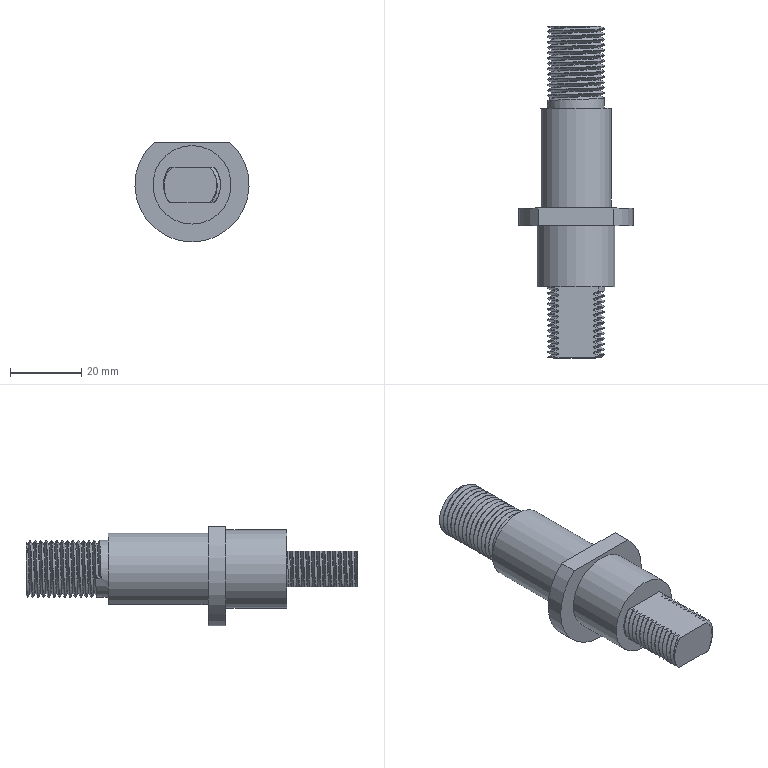Component | NX | LOCATING_PEG | 1 solid | 136 faces | volume 25845 mm3 | cylinder 71 | spline 55 | plane 10 | commonest cylinder face diameters 16 x41 14 x27 22 x1 32 x1 20 x1